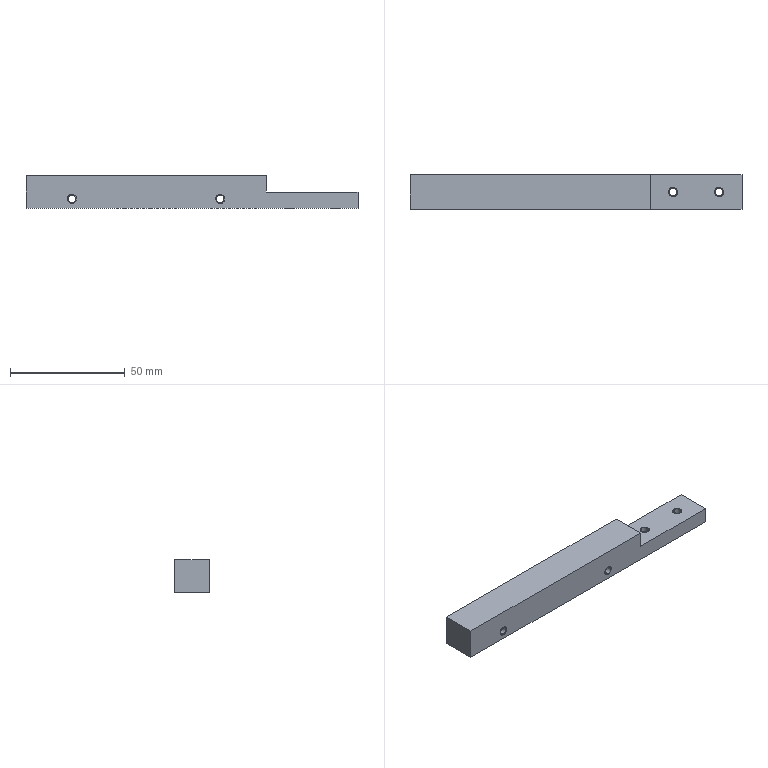CAM job | Mastercam | mm | 11 operations | part box 144.5 x 15 x 14
1. Facing | 12 - 12 平铣刀
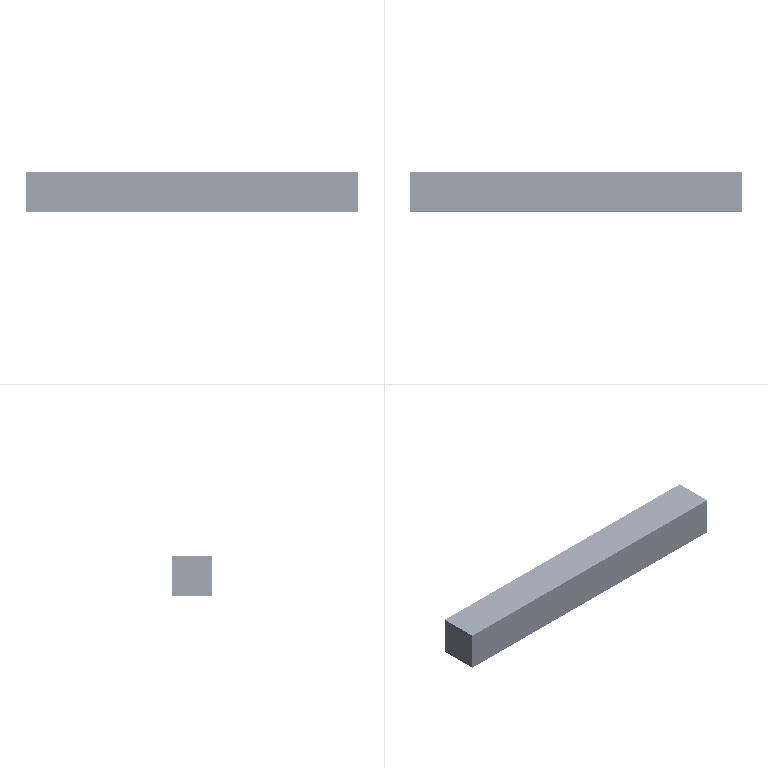2. 2D High Speed (2D Dynamic Mill) | 12 - 12 平铣刀
3. Contour (2D) | 12 - 12 平铣刀
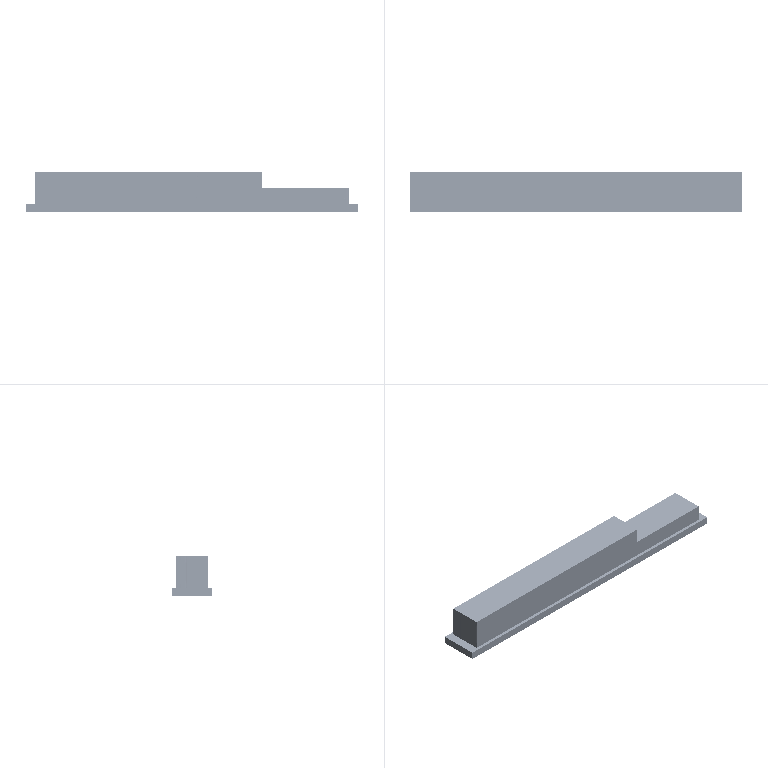4. Contour (2D) | 12 - 12 平铣刀
5. Contour (2D) | 12 - 12 平铣刀
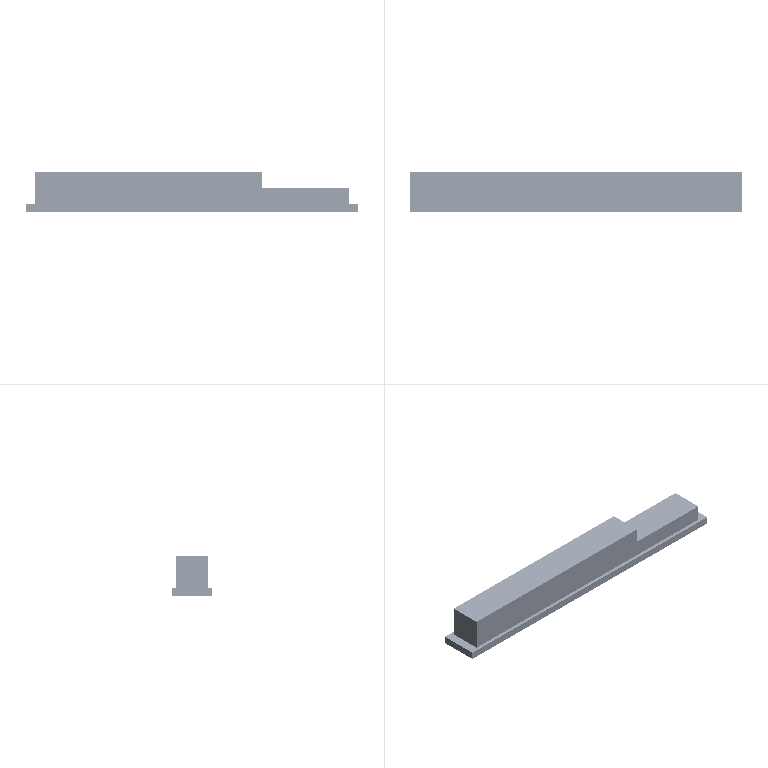6. Model Chamfer | 7 - 4 倒角刀
7. Drill/Counterbore | 7 - 4 倒角刀
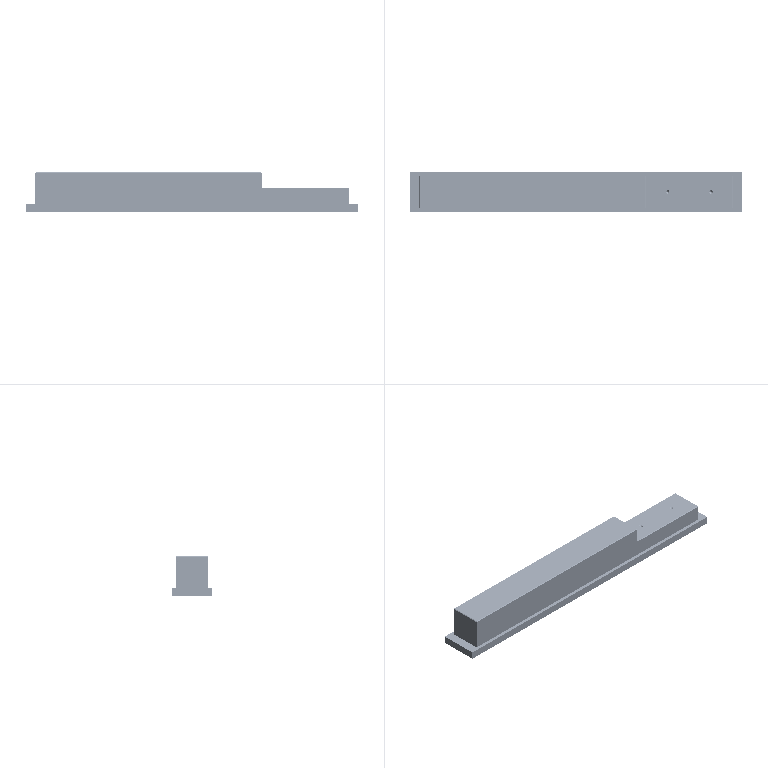8. Facing | 12 - 12 平铣刀
9. Facing | 6 - 6 平铣刀
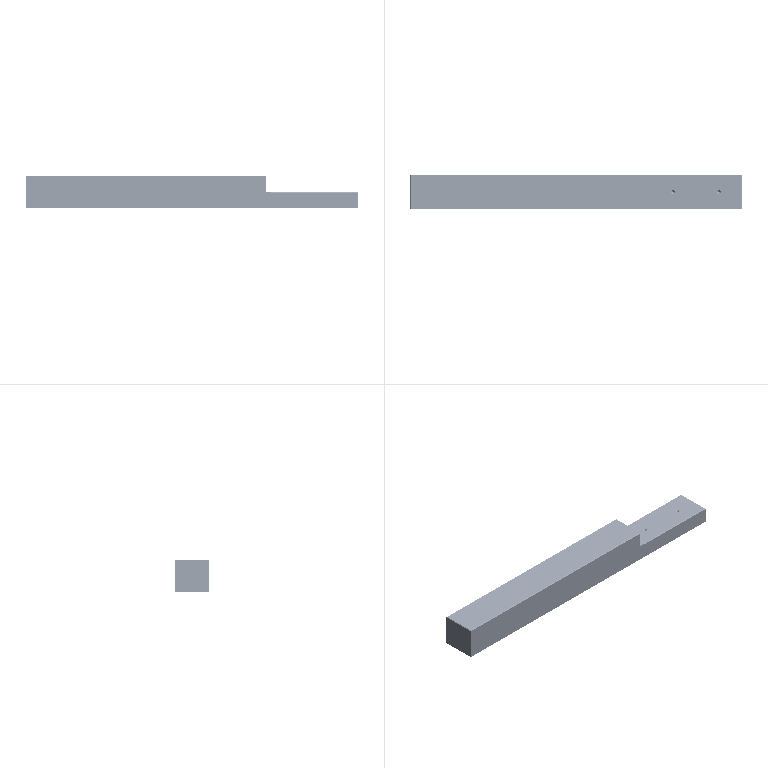10. Contour (2D chamfer) | 7 - 4 倒角刀
11. Drill/Counterbore | 7 - 4 倒角刀